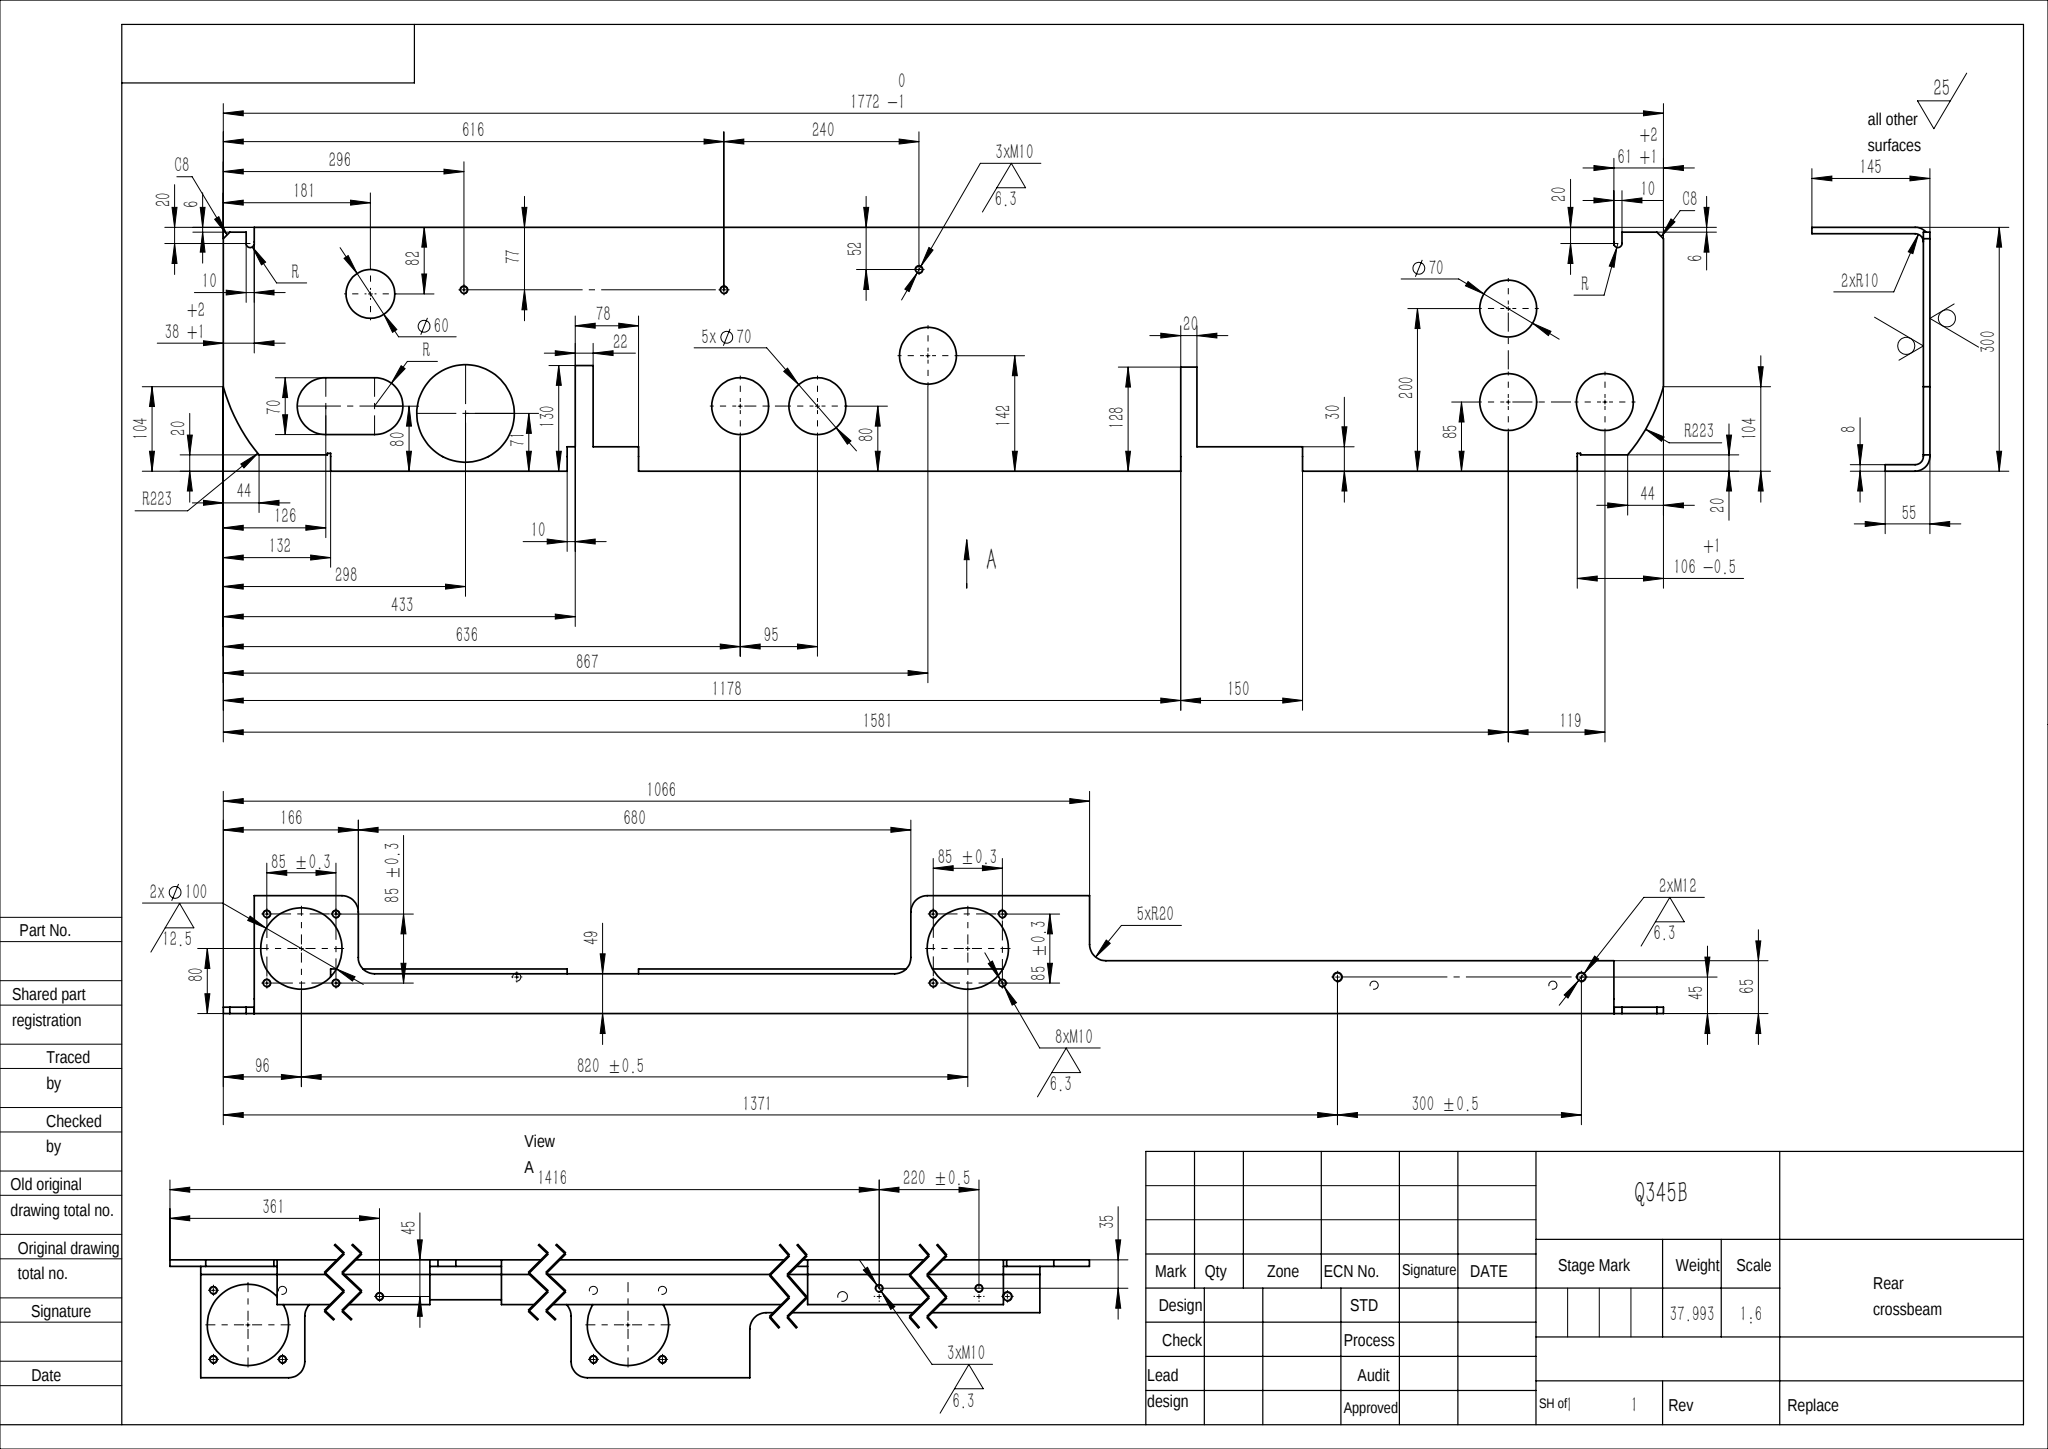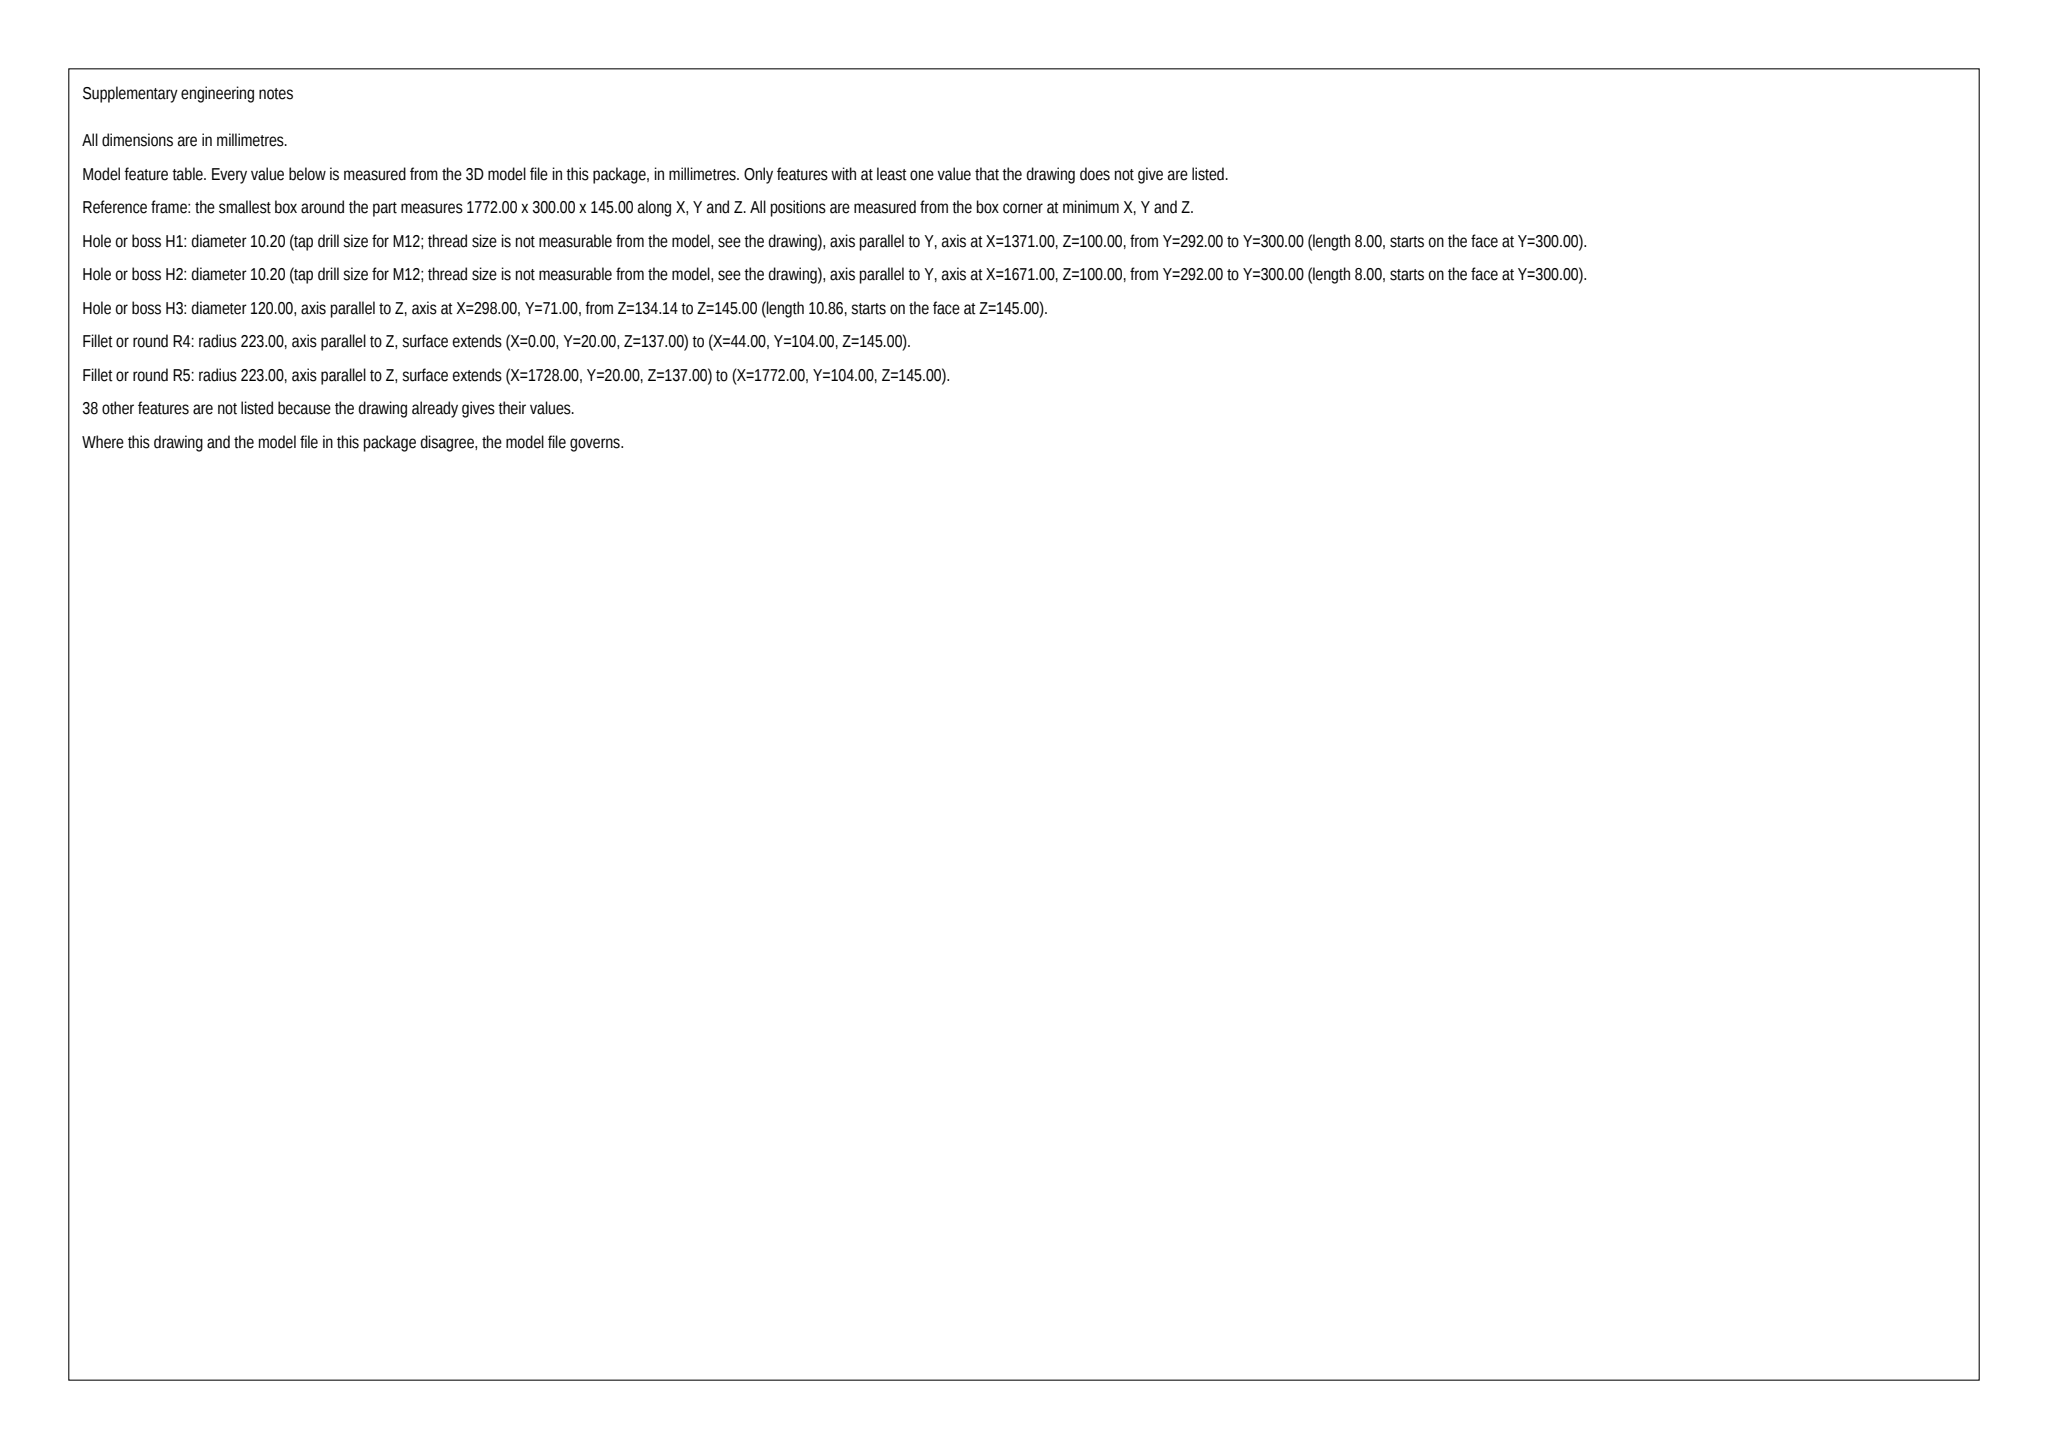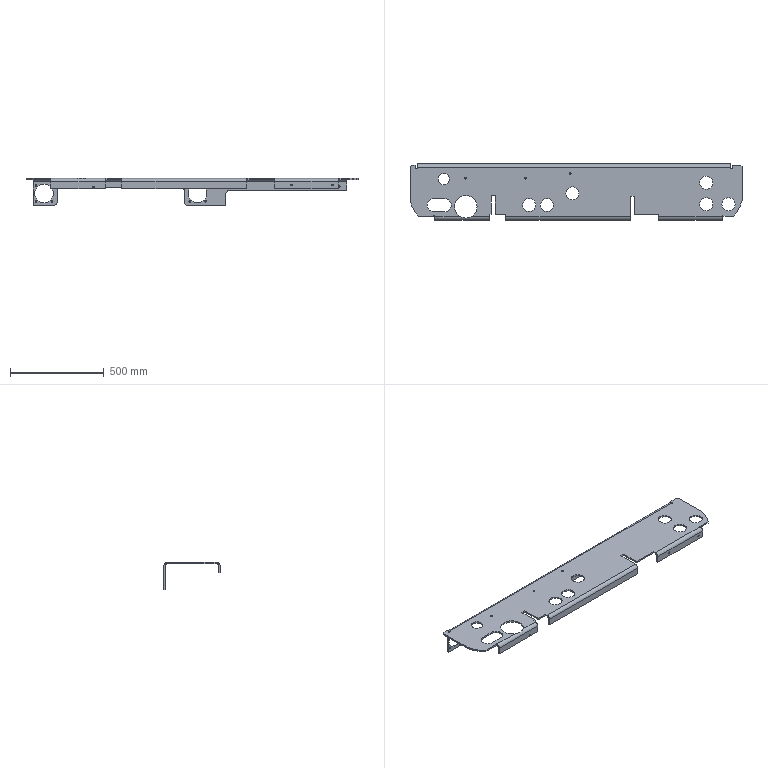Part | SolidWorks | mm | material Q345B | 1 solid | 140 faces | box 1772 x 300 x 145 mm | volume 4839872 mm3 | cylinder 72 | plane 68 | commonest cylinder face diameters 8.5 x28 70 x15 40 x5 10.2 x4 100 x4 36 x4 20 x4 120 x2